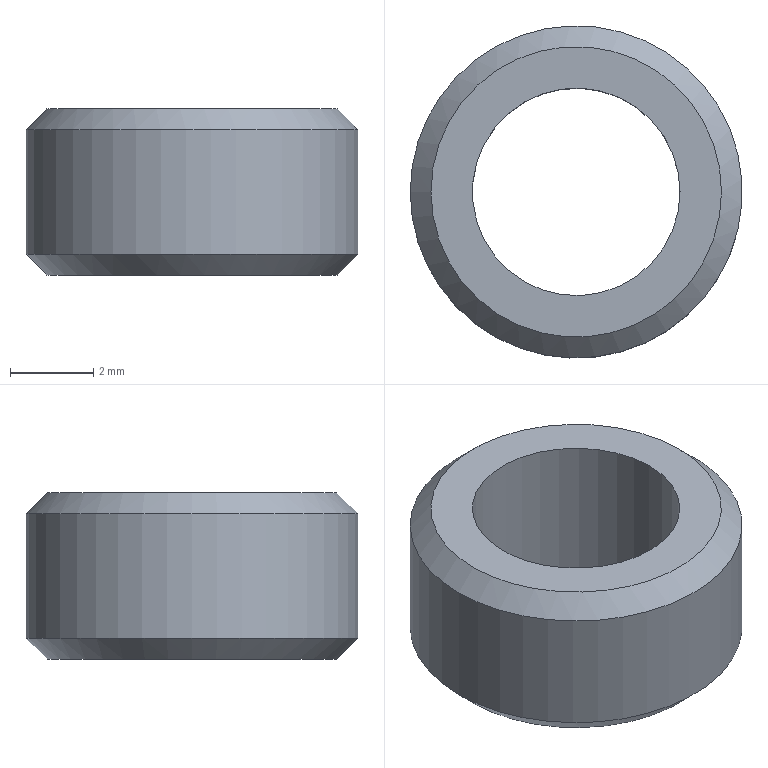Component | NX | NUT | 1 solid | 6 faces | box 8 x 8 x 4 mm | volume 117 mm3 | cylinder 2 | plane 2 | cone 2 | commonest cylinder face diameters 8 x1 5 x1
STEP:
#1=CARTESIAN_POINT('',(0.,0.,0.));
#2=DIRECTION('',(0.,0.,1.));
#3=DIRECTION('',(1.,0.,0.));
#4=AXIS2_PLACEMENT_3D('',#1,#2,#3);
#5=CARTESIAN_POINT('',(-25.665,0.,8.5));
#6=VERTEX_POINT('',#5);
#7=CARTESIAN_POINT('',(-21.665,0.,8.5));
#8=DIRECTION('',(0.,0.,1.));
#9=DIRECTION('',(-1.,0.,0.));
#10=AXIS2_PLACEMENT_3D('',#7,#8,#9);
#11=CIRCLE('',#10,4.);
#12=CARTESIAN_POINT('',(-21.665,0.,12.));
#13=DIRECTION('',(0.,0.,-1.));
#14=DIRECTION('',(-1.,0.,0.));
#15=AXIS2_PLACEMENT_3D('',#12,#13,#14);
#16=CYLINDRICAL_SURFACE('',#15,4.);
#17=CARTESIAN_POINT('',(6.283,3.5));
#18=DIRECTION('',(-1.,0.));
#19=VECTOR('',#18,1.);
#20=LINE('',#17,#19);
#21=(GEOMETRIC_REPRESENTATION_CONTEXT(2)PARAMETRIC_REPRESENTATION_CONTEXT()REPRESENTATION_CONTEXT('',''));
#22=DEFINITIONAL_REPRESENTATION('',(#20),#21);
#23=PCURVE('',#16,#22);
#24=CARTESIAN_POINT('',(-21.665,0.,8.));
#25=DIRECTION('',(0.,0.,1.));
#26=DIRECTION('',(1.,0.,0.));
#27=AXIS2_PLACEMENT_3D('',#24,#25,#26);
#28=CONICAL_SURFACE('',#27,3.5,0.7854);
#29=CARTESIAN_POINT('',(3.142,0.5));
#30=DIRECTION('',(1.,0.));
#31=VECTOR('',#30,1.);
#32=LINE('',#29,#31);
#33=(GEOMETRIC_REPRESENTATION_CONTEXT(2)PARAMETRIC_REPRESENTATION_CONTEXT()REPRESENTATION_CONTEXT('',''));
#34=DEFINITIONAL_REPRESENTATION('',(#32),#33);
#35=PCURVE('',#28,#34);
#36=SURFACE_CURVE('',#11,(#23,#35),.PCURVE_S1.);
#37=EDGE_CURVE('',#6,#6,#36,.T.);
#38=ORIENTED_EDGE('',*,*,#37,.T.);
#39=CARTESIAN_POINT('',(-25.665,0.,11.5));
#40=VERTEX_POINT('',#39);
#41=CARTESIAN_POINT('',(-25.665,-0.,11.5));
#42=CARTESIAN_POINT('',(-25.665,-0.,8.5));
#43=B_SPLINE_CURVE_WITH_KNOTS('',1,(#41,#42),.UNSPECIFIED.,.F.,.F.,(2,2),(0.5,3.5),.PIECEWISE_BEZIER_KNOTS.);
#44=CARTESIAN_POINT('',(0.,0.));
#45=DIRECTION('',(0.,1.));
#46=VECTOR('',#45,1.);
#47=LINE('',#44,#46);
#48=(GEOMETRIC_REPRESENTATION_CONTEXT(2)PARAMETRIC_REPRESENTATION_CONTEXT()REPRESENTATION_CONTEXT('',''));
#49=DEFINITIONAL_REPRESENTATION('',(#47),#48);
#50=PCURVE('',#16,#49);
#51=CARTESIAN_POINT('',(6.283,0.));
#52=DIRECTION('',(0.,1.));
#53=VECTOR('',#52,1.);
#54=LINE('',#51,#53);
#55=(GEOMETRIC_REPRESENTATION_CONTEXT(2)PARAMETRIC_REPRESENTATION_CONTEXT()REPRESENTATION_CONTEXT('',''));
#56=DEFINITIONAL_REPRESENTATION('',(#54),#55);
#57=PCURVE('',#16,#56);
#58=SEAM_CURVE('',#43,(#50,#57),.PCURVE_S1.);
#59=EDGE_CURVE('',#40,#6,#58,.T.);
#60=ORIENTED_EDGE('',*,*,#59,.F.);
#61=CARTESIAN_POINT('',(-21.665,0.,11.5));
#62=DIRECTION('',(0.,0.,-1.));
#63=DIRECTION('',(-1.,0.,0.));
#64=AXIS2_PLACEMENT_3D('',#61,#62,#63);
#65=CIRCLE('',#64,4.);
#66=CARTESIAN_POINT('',(0.,0.5));
#67=DIRECTION('',(1.,0.));
#68=VECTOR('',#67,1.);
#69=LINE('',#66,#68);
#70=(GEOMETRIC_REPRESENTATION_CONTEXT(2)PARAMETRIC_REPRESENTATION_CONTEXT()REPRESENTATION_CONTEXT('',''));
#71=DEFINITIONAL_REPRESENTATION('',(#69),#70);
#72=PCURVE('',#16,#71);
#73=CARTESIAN_POINT('',(-21.665,0.,11.5));
#74=DIRECTION('',(0.,0.,-1.));
#75=DIRECTION('',(-1.,0.,0.));
#76=AXIS2_PLACEMENT_3D('',#73,#74,#75);
#77=CONICAL_SURFACE('',#76,4.,0.7854);
#78=CARTESIAN_POINT('',(0.,0.));
#79=DIRECTION('',(1.,0.));
#80=VECTOR('',#79,1.);
#81=LINE('',#78,#80);
#82=(GEOMETRIC_REPRESENTATION_CONTEXT(2)PARAMETRIC_REPRESENTATION_CONTEXT()REPRESENTATION_CONTEXT('',''));
#83=DEFINITIONAL_REPRESENTATION('',(#81),#82);
#84=PCURVE('',#77,#83);
#85=SURFACE_CURVE('',#65,(#72,#84),.PCURVE_S1.);
#86=EDGE_CURVE('',#40,#40,#85,.T.);
#87=ORIENTED_EDGE('',*,*,#86,.T.);
#88=ORIENTED_EDGE('',*,*,#59,.T.);
#89=EDGE_LOOP('',(#38,#60,#87,#88));
#90=FACE_BOUND('',#89,.T.);
#91=ADVANCED_FACE('',(#90),#16,.T.);
#92=CARTESIAN_POINT('',(-19.165,0.,12.));
#93=VERTEX_POINT('',#92);
#94=CARTESIAN_POINT('',(-21.665,0.,12.));
#95=DIRECTION('',(0.,0.,-1.));
#96=DIRECTION('',(1.,0.,0.));
#97=AXIS2_PLACEMENT_3D('',#94,#95,#96);
#98=CIRCLE('',#97,2.5);
#99=CARTESIAN_POINT('',(-21.665,0.,12.));
#100=DIRECTION('',(0.,0.,-1.));
#101=DIRECTION('',(-1.,0.,0.));
#102=AXIS2_PLACEMENT_3D('',#99,#100,#101);
#103=CYLINDRICAL_SURFACE('',#102,2.5);
#104=CARTESIAN_POINT('',(3.142,0.));
#105=DIRECTION('',(1.,0.));
#106=VECTOR('',#105,1.);
#107=LINE('',#104,#106);
#108=(GEOMETRIC_REPRESENTATION_CONTEXT(2)PARAMETRIC_REPRESENTATION_CONTEXT()REPRESENTATION_CONTEXT('',''));
#109=DEFINITIONAL_REPRESENTATION('',(#107),#108);
#110=PCURVE('',#103,#109);
#111=CARTESIAN_POINT('',(-21.665,0.,12.));
#112=DIRECTION('',(0.,0.,-1.));
#113=DIRECTION('',(-1.,0.,0.));
#114=AXIS2_PLACEMENT_3D('',#111,#112,#113);
#115=PLANE('',#114);
#116=CARTESIAN_POINT('',(0.,0.));
#117=DIRECTION('',(-1.,0.));
#118=AXIS2_PLACEMENT_2D('',#116,#117);
#119=CIRCLE('',#118,2.5);
#120=(GEOMETRIC_REPRESENTATION_CONTEXT(2)PARAMETRIC_REPRESENTATION_CONTEXT()REPRESENTATION_CONTEXT('',''));
#121=DEFINITIONAL_REPRESENTATION('',(#119),#120);
#122=PCURVE('',#115,#121);
#123=SURFACE_CURVE('',#98,(#110,#122),.PCURVE_S1.);
#124=EDGE_CURVE('',#93,#93,#123,.T.);
#125=ORIENTED_EDGE('',*,*,#124,.T.);
#126=CARTESIAN_POINT('',(-19.165,0.,8.));
#127=VERTEX_POINT('',#126);
#128=CARTESIAN_POINT('',(-19.165,0.,12.));
#129=CARTESIAN_POINT('',(-19.165,0.,8.));
#130=B_SPLINE_CURVE_WITH_KNOTS('',1,(#128,#129),.UNSPECIFIED.,.F.,.F.,(2,2),(0.,4.),.PIECEWISE_BEZIER_KNOTS.);
#131=CARTESIAN_POINT('',(9.425,0.));
#132=DIRECTION('',(0.,1.));
#133=VECTOR('',#132,1.);
#134=LINE('',#131,#133);
#135=(GEOMETRIC_REPRESENTATION_CONTEXT(2)PARAMETRIC_REPRESENTATION_CONTEXT()REPRESENTATION_CONTEXT('',''));
#136=DEFINITIONAL_REPRESENTATION('',(#134),#135);
#137=PCURVE('',#103,#136);
#138=CARTESIAN_POINT('',(3.142,0.));
#139=DIRECTION('',(0.,1.));
#140=VECTOR('',#139,1.);
#141=LINE('',#138,#140);
#142=(GEOMETRIC_REPRESENTATION_CONTEXT(2)PARAMETRIC_REPRESENTATION_CONTEXT()REPRESENTATION_CONTEXT('',''));
#143=DEFINITIONAL_REPRESENTATION('',(#141),#142);
#144=PCURVE('',#103,#143);
#145=SEAM_CURVE('',#130,(#137,#144),.PCURVE_S1.);
#146=EDGE_CURVE('',#93,#127,#145,.T.);
#147=ORIENTED_EDGE('',*,*,#146,.T.);
#148=CARTESIAN_POINT('',(-21.665,0.,8.));
#149=DIRECTION('',(0.,0.,-1.));
#150=DIRECTION('',(1.,0.,0.));
#151=AXIS2_PLACEMENT_3D('',#148,#149,#150);
#152=CIRCLE('',#151,2.5);
#153=CARTESIAN_POINT('',(3.142,4.));
#154=DIRECTION('',(1.,0.));
#155=VECTOR('',#154,1.);
#156=LINE('',#153,#155);
#157=(GEOMETRIC_REPRESENTATION_CONTEXT(2)PARAMETRIC_REPRESENTATION_CONTEXT()REPRESENTATION_CONTEXT('',''));
#158=DEFINITIONAL_REPRESENTATION('',(#156),#157);
#159=PCURVE('',#103,#158);
#160=CARTESIAN_POINT('',(-21.665,0.,8.));
#161=DIRECTION('',(0.,0.,-1.));
#162=DIRECTION('',(-1.,0.,0.));
#163=AXIS2_PLACEMENT_3D('',#160,#161,#162);
#164=PLANE('',#163);
#165=CARTESIAN_POINT('',(0.,0.));
#166=DIRECTION('',(-1.,0.));
#167=AXIS2_PLACEMENT_2D('',#165,#166);
#168=CIRCLE('',#167,2.5);
#169=(GEOMETRIC_REPRESENTATION_CONTEXT(2)PARAMETRIC_REPRESENTATION_CONTEXT()REPRESENTATION_CONTEXT('',''));
#170=DEFINITIONAL_REPRESENTATION('',(#168),#169);
#171=PCURVE('',#164,#170);
#172=SURFACE_CURVE('',#152,(#159,#171),.PCURVE_S1.);
#173=EDGE_CURVE('',#127,#127,#172,.T.);
#174=ORIENTED_EDGE('',*,*,#173,.F.);
#175=ORIENTED_EDGE('',*,*,#146,.F.);
#176=EDGE_LOOP('',(#125,#147,#174,#175));
#177=FACE_BOUND('',#176,.F.);
#178=ADVANCED_FACE('',(#177),#103,.F.);
#179=CARTESIAN_POINT('',(-25.165,0.,12.));
#180=VERTEX_POINT('',#179);
#181=CARTESIAN_POINT('',(-21.665,0.,12.));
#182=DIRECTION('',(0.,0.,1.));
#183=DIRECTION('',(-1.,0.,0.));
#184=AXIS2_PLACEMENT_3D('',#181,#182,#183);
#185=CIRCLE('',#184,3.5);
#186=CARTESIAN_POINT('',(3.5,0.));
#187=CARTESIAN_POINT('',(3.5,-6.062));
#188=CARTESIAN_POINT('',(-1.75,-3.031));
#189=CARTESIAN_POINT('',(-7.,-0.));
#190=CARTESIAN_POINT('',(-1.75,3.031));
#191=CARTESIAN_POINT('',(3.5,6.062));
#192=CARTESIAN_POINT('',(3.5,0.));
#193=(BOUNDED_CURVE()B_SPLINE_CURVE(2,(#186,#187,#188,#189,#190,#191,#192),.UNSPECIFIED.,.T.,.F.)B_SPLINE_CURVE_WITH_KNOTS((1,2,2,2,2,1),(-2.094,0.,2.094,4.189,6.283,8.378),.UNSPECIFIED.)CURVE()GEOMETRIC_REPRESENTATION_ITEM()RATIONAL_B_SPLINE_CURVE((1.,0.5,1.,0.5,1.,0.5,1.))REPRESENTATION_ITEM(''));
#194=(GEOMETRIC_REPRESENTATION_CONTEXT(2)PARAMETRIC_REPRESENTATION_CONTEXT()REPRESENTATION_CONTEXT('',''));
#195=DEFINITIONAL_REPRESENTATION('',(#193),#194);
#196=PCURVE('',#115,#195);
#197=CARTESIAN_POINT('',(6.283,-0.5));
#198=DIRECTION('',(-1.,0.));
#199=VECTOR('',#198,1.);
#200=LINE('',#197,#199);
#201=(GEOMETRIC_REPRESENTATION_CONTEXT(2)PARAMETRIC_REPRESENTATION_CONTEXT()REPRESENTATION_CONTEXT('',''));
#202=DEFINITIONAL_REPRESENTATION('',(#200),#201);
#203=PCURVE('',#77,#202);
#204=SURFACE_CURVE('',#185,(#196,#203),.PCURVE_S1.);
#205=EDGE_CURVE('',#180,#180,#204,.T.);
#206=ORIENTED_EDGE('',*,*,#205,.T.);
#207=EDGE_LOOP('',(#206));
#208=FACE_BOUND('',#207,.T.);
#209=ORIENTED_EDGE('',*,*,#124,.T.);
#210=EDGE_LOOP('',(#209));
#211=FACE_BOUND('',#210,.T.);
#212=ADVANCED_FACE('',(#208,#211),#115,.F.);
#213=CARTESIAN_POINT('',(-25.165,0.,8.));
#214=VERTEX_POINT('',#213);
#215=CARTESIAN_POINT('',(-21.665,0.,8.));
#216=DIRECTION('',(0.,0.,-1.));
#217=DIRECTION('',(-1.,0.,0.));
#218=AXIS2_PLACEMENT_3D('',#215,#216,#217);
#219=CIRCLE('',#218,3.5);
#220=CARTESIAN_POINT('',(0.,0.));
#221=DIRECTION('',(1.,0.));
#222=AXIS2_PLACEMENT_2D('',#220,#221);
#223=CIRCLE('',#222,3.5);
#224=(GEOMETRIC_REPRESENTATION_CONTEXT(2)PARAMETRIC_REPRESENTATION_CONTEXT()REPRESENTATION_CONTEXT('',''));
#225=DEFINITIONAL_REPRESENTATION('',(#223),#224);
#226=PCURVE('',#164,#225);
#227=CARTESIAN_POINT('',(9.425,0.));
#228=DIRECTION('',(-1.,0.));
#229=VECTOR('',#228,1.);
#230=LINE('',#227,#229);
#231=(GEOMETRIC_REPRESENTATION_CONTEXT(2)PARAMETRIC_REPRESENTATION_CONTEXT()REPRESENTATION_CONTEXT('',''));
#232=DEFINITIONAL_REPRESENTATION('',(#230),#231);
#233=PCURVE('',#28,#232);
#234=SURFACE_CURVE('',#219,(#226,#233),.PCURVE_S1.);
#235=EDGE_CURVE('',#214,#214,#234,.T.);
#236=ORIENTED_EDGE('',*,*,#235,.T.);
#237=EDGE_LOOP('',(#236));
#238=FACE_BOUND('',#237,.T.);
#239=ORIENTED_EDGE('',*,*,#173,.F.);
#240=EDGE_LOOP('',(#239));
#241=FACE_BOUND('',#240,.T.);
#242=ADVANCED_FACE('',(#238,#241),#164,.T.);
#243=ORIENTED_EDGE('',*,*,#37,.F.);
#244=CARTESIAN_POINT('',(-25.165,0.,8.));
#245=CARTESIAN_POINT('',(-25.665,0.,8.5));
#246=B_SPLINE_CURVE_WITH_KNOTS('',1,(#244,#245),.UNSPECIFIED.,.F.,.F.,(2,2),(0.,0.7071),.PIECEWISE_BEZIER_KNOTS.);
#247=CARTESIAN_POINT('',(3.142,0.));
#248=DIRECTION('',(0.,1.));
#249=VECTOR('',#248,1.);
#250=LINE('',#247,#249);
#251=(GEOMETRIC_REPRESENTATION_CONTEXT(2)PARAMETRIC_REPRESENTATION_CONTEXT()REPRESENTATION_CONTEXT('',''));
#252=DEFINITIONAL_REPRESENTATION('',(#250),#251);
#253=PCURVE('',#28,#252);
#254=CARTESIAN_POINT('',(9.425,0.));
#255=DIRECTION('',(0.,1.));
#256=VECTOR('',#255,1.);
#257=LINE('',#254,#256);
#258=(GEOMETRIC_REPRESENTATION_CONTEXT(2)PARAMETRIC_REPRESENTATION_CONTEXT()REPRESENTATION_CONTEXT('',''));
#259=DEFINITIONAL_REPRESENTATION('',(#257),#258);
#260=PCURVE('',#28,#259);
#261=SEAM_CURVE('',#246,(#253,#260),.PCURVE_S1.);
#262=EDGE_CURVE('',#214,#6,#261,.T.);
#263=ORIENTED_EDGE('',*,*,#262,.F.);
#264=ORIENTED_EDGE('',*,*,#235,.F.);
#265=ORIENTED_EDGE('',*,*,#262,.T.);
#266=EDGE_LOOP('',(#243,#263,#264,#265));
#267=FACE_BOUND('',#266,.T.);
#268=ADVANCED_FACE('',(#267),#28,.T.);
#269=ORIENTED_EDGE('',*,*,#205,.F.);
#270=CARTESIAN_POINT('',(-25.165,0.,12.));
#271=CARTESIAN_POINT('',(-25.665,0.,11.5));
#272=B_SPLINE_CURVE_WITH_KNOTS('',1,(#270,#271),.UNSPECIFIED.,.F.,.F.,(2,2),(-0.7071,0.),.PIECEWISE_BEZIER_KNOTS.);
#273=CARTESIAN_POINT('',(6.283,0.));
#274=DIRECTION('',(0.,1.));
#275=VECTOR('',#274,1.);
#276=LINE('',#273,#275);
#277=(GEOMETRIC_REPRESENTATION_CONTEXT(2)PARAMETRIC_REPRESENTATION_CONTEXT()REPRESENTATION_CONTEXT('',''));
#278=DEFINITIONAL_REPRESENTATION('',(#276),#277);
#279=PCURVE('',#77,#278);
#280=CARTESIAN_POINT('',(0.,0.));
#281=DIRECTION('',(0.,1.));
#282=VECTOR('',#281,1.);
#283=LINE('',#280,#282);
#284=(GEOMETRIC_REPRESENTATION_CONTEXT(2)PARAMETRIC_REPRESENTATION_CONTEXT()REPRESENTATION_CONTEXT('',''));
#285=DEFINITIONAL_REPRESENTATION('',(#283),#284);
#286=PCURVE('',#77,#285);
#287=SEAM_CURVE('',#272,(#279,#286),.PCURVE_S1.);
#288=EDGE_CURVE('',#180,#40,#287,.T.);
#289=ORIENTED_EDGE('',*,*,#288,.T.);
#290=ORIENTED_EDGE('',*,*,#86,.F.);
#291=ORIENTED_EDGE('',*,*,#288,.F.);
#292=EDGE_LOOP('',(#269,#289,#290,#291));
#293=FACE_BOUND('',#292,.T.);
#294=ADVANCED_FACE('',(#293),#77,.T.);
#295=CLOSED_SHELL('',(#91,#178,#212,#242,#268,#294));
#296=MANIFOLD_SOLID_BREP('',#295);
#297=(LENGTH_UNIT()NAMED_UNIT(*)SI_UNIT(.MILLI.,.METRE.));
#298=UNCERTAINTY_MEASURE_WITH_UNIT(LENGTH_MEASURE(0.00001),#297,'','');
#299=(NAMED_UNIT(*)PLANE_ANGLE_UNIT()SI_UNIT($,.RADIAN.));
#300=(NAMED_UNIT(*)SI_UNIT($,.STERADIAN.)SOLID_ANGLE_UNIT());
#301=(GEOMETRIC_REPRESENTATION_CONTEXT(3)GLOBAL_UNCERTAINTY_ASSIGNED_CONTEXT((#298))GLOBAL_UNIT_ASSIGNED_CONTEXT((#297,#299,#300))REPRESENTATION_CONTEXT('',''));
#302=ADVANCED_BREP_SHAPE_REPRESENTATION('',(#4,#296),#301);